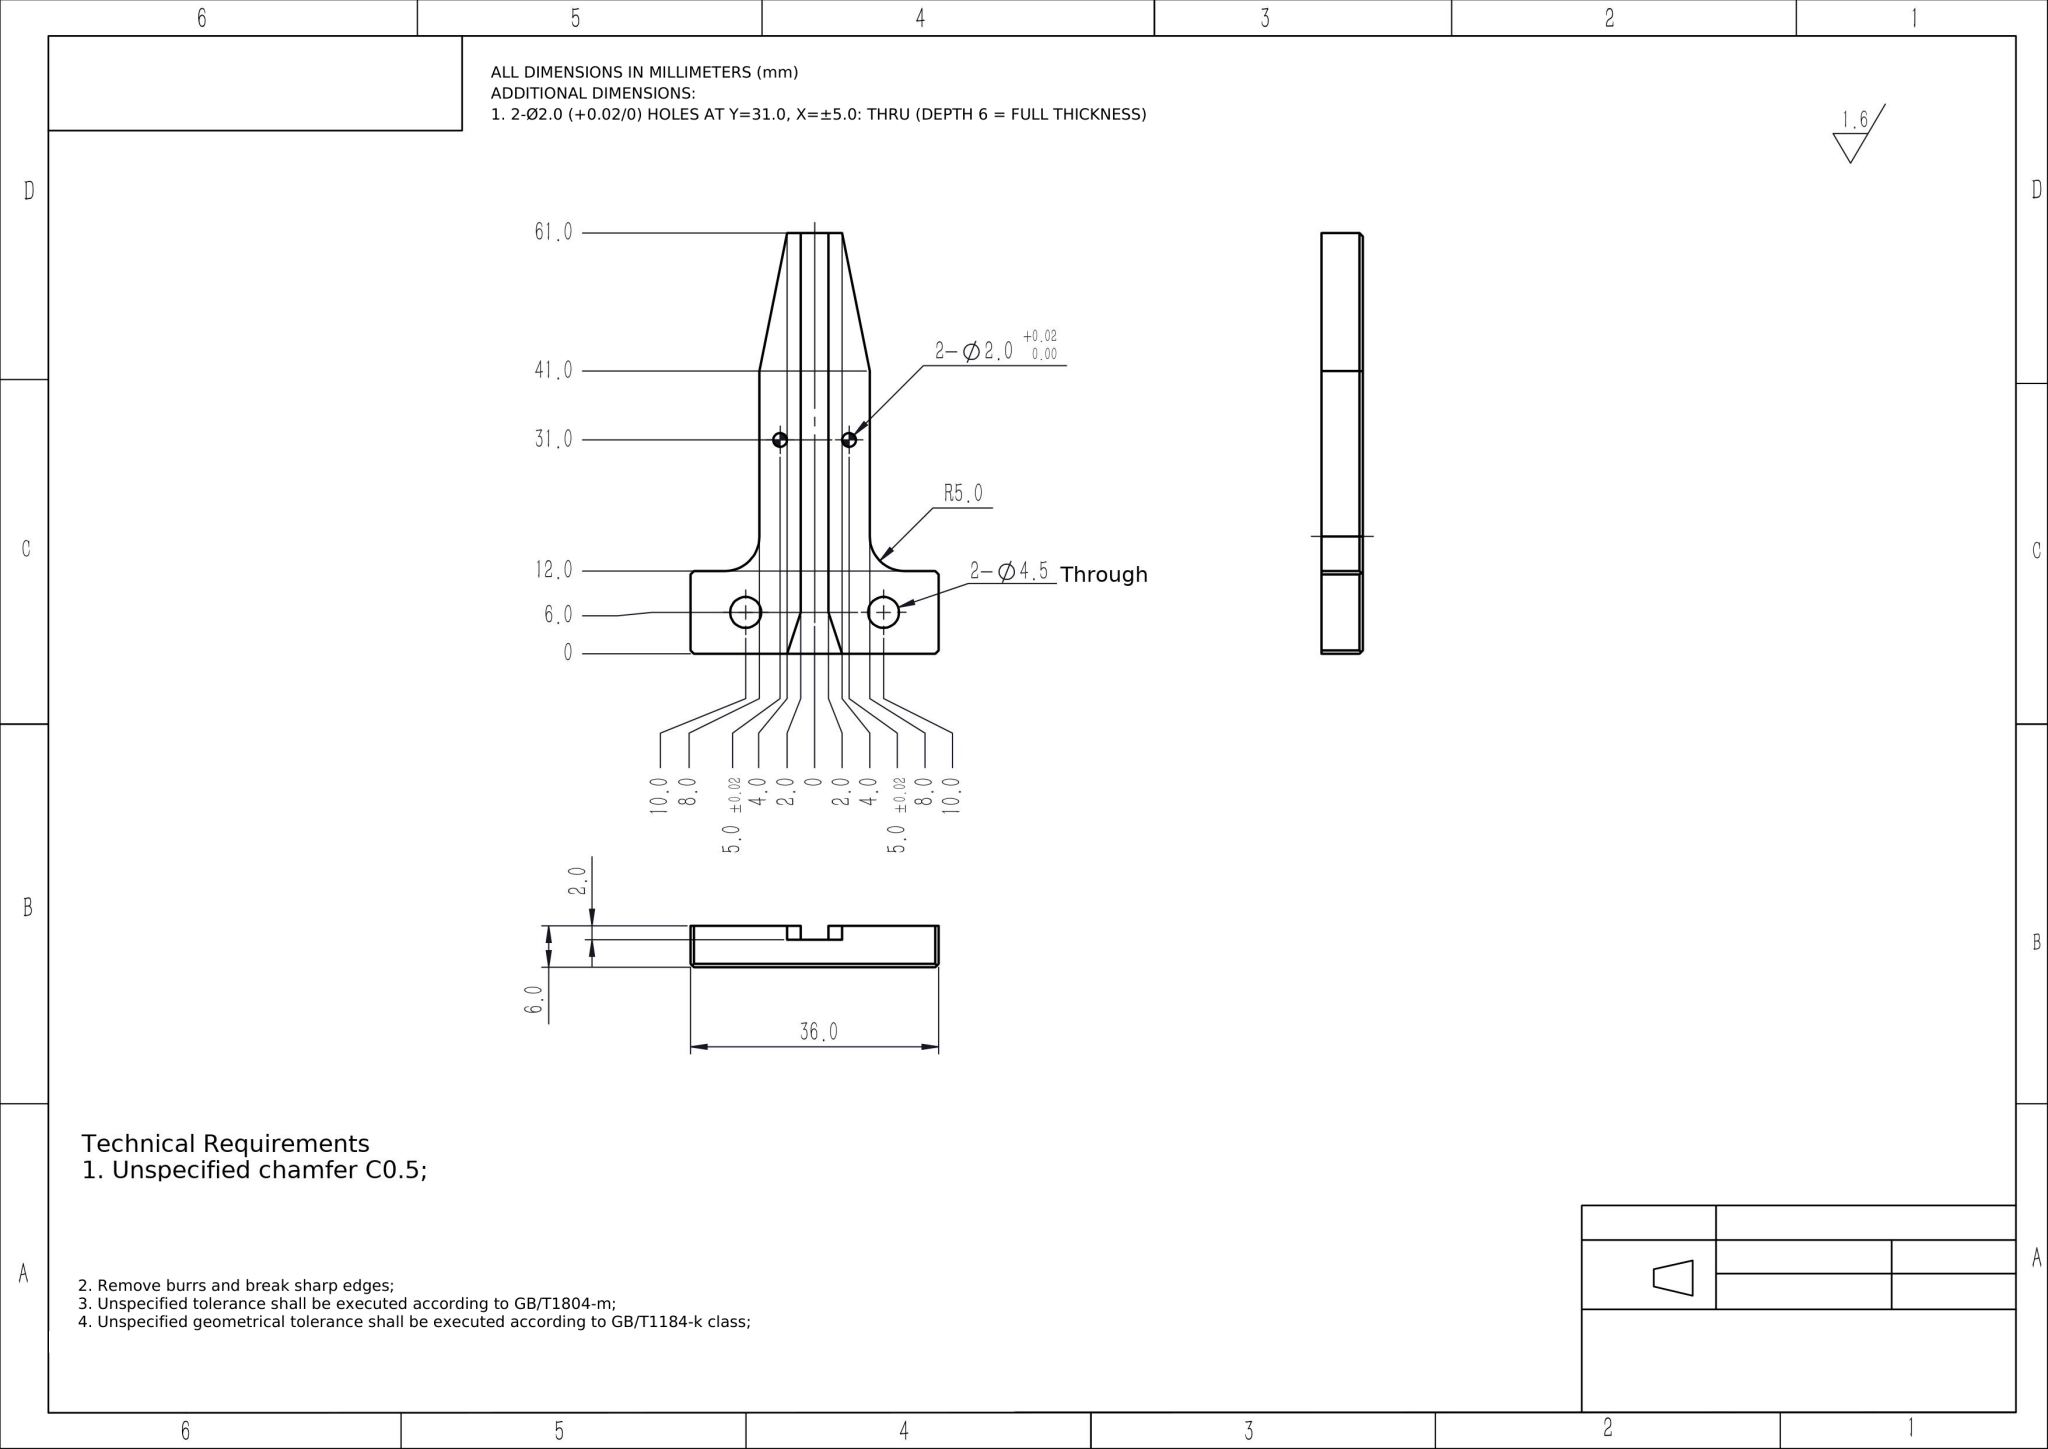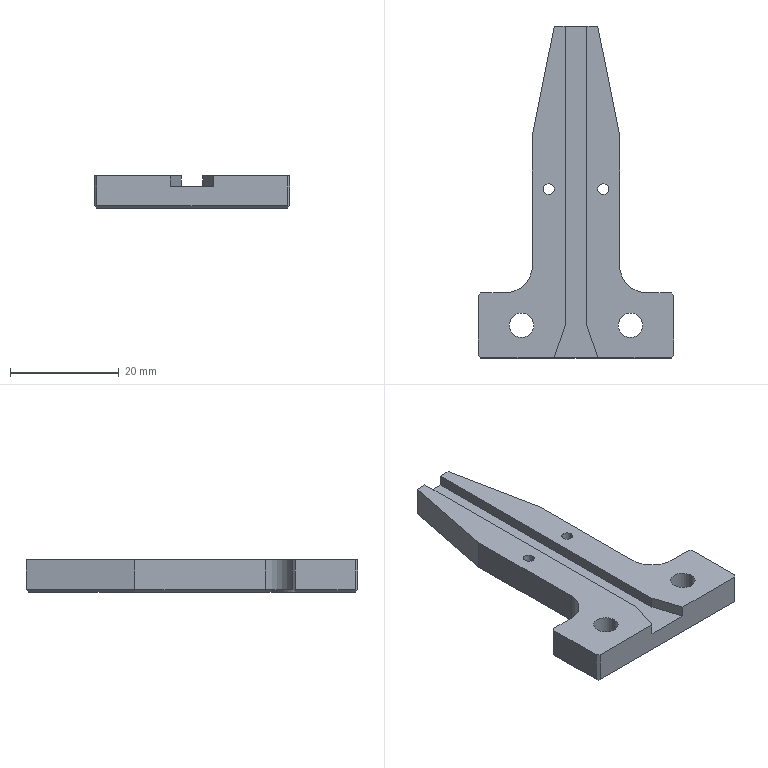Part | NX | mm | 1 solid | 44 faces | box 36 x 61 x 6 mm | volume 6114 mm3 | plane 32 | cylinder 10 | cone 2 | commonest cylinder face diameters 2 x4 4.5 x4 10 x2